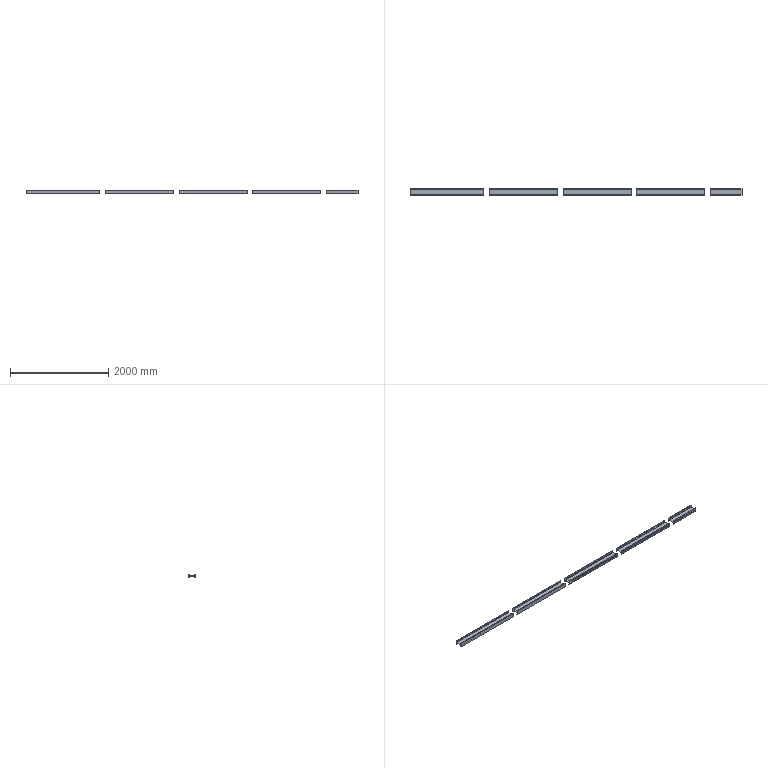Component | NX | FUGUJIA | 5 solids | 90 faces | volume 13682149 mm3 | plane 70 | cylinder 20 | commonest cylinder face diameters 15 x20